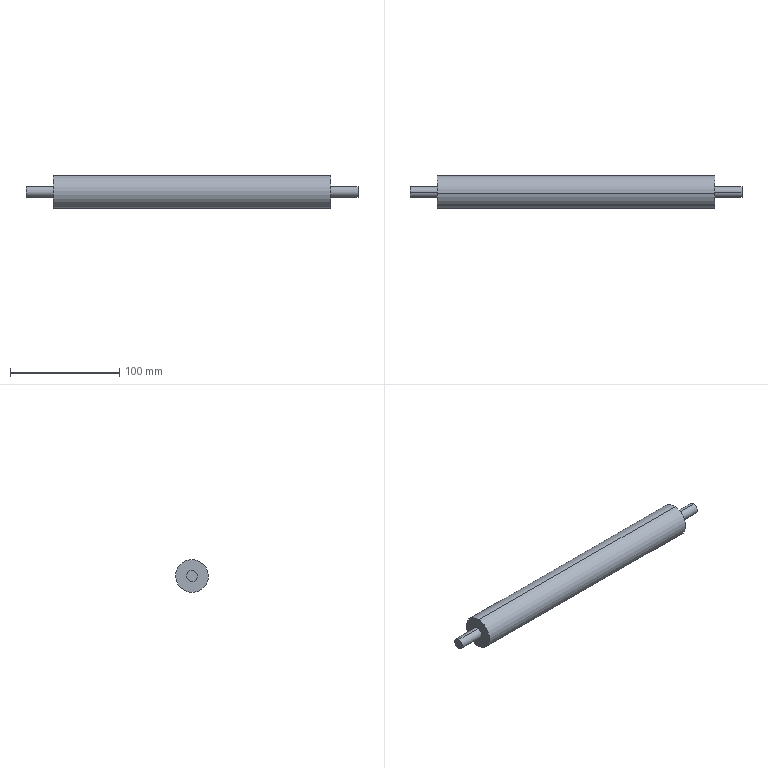Component | SolidWorks | Part5-1 | 1 solid | 10 faces | box 304 x 30 x 30 mm | volume 183469 mm3 | cylinder 6 | plane 4 | commonest cylinder face diameters 10 x4 30 x2
build123d program:
from build123d import *

# Parameters (mm, degrees)
SKETCH1_R           = 5
BOSS_EXTRUDE1_DEPTH = 152
SKETCH2_R           = 15
BOSS_EXTRUDE2_DEPTH = 127


with BuildPart() as part:
    # Sketch1 → Boss-Extrude1 (new, symmetric)
    with BuildSketch(Plane.XY):
        with Locations((-94.809, 415)):
            Circle(SKETCH1_R)
    extrude(amount=BOSS_EXTRUDE1_DEPTH, both=True)

    # Sketch2 → Boss-Extrude2 (add, symmetric)
    with BuildSketch(Plane.XY):
        with Locations((-94.809, 415)):
            Circle(SKETCH2_R)
    extrude(amount=BOSS_EXTRUDE2_DEPTH, both=True)


solid = part.part

# Placed as in the assembly
solid = solid.moved(Location((0, 0, -210.206), (0, 90, 0)))
STEP:
#1=COLOUR_RGB('',0.7922,0.8196,0.9333);
#2=FILL_AREA_STYLE_COLOUR('',#1);
#3=FILL_AREA_STYLE('',(#2));
#4=SURFACE_STYLE_FILL_AREA(#3);
#5=SURFACE_SIDE_STYLE('',(#4));
#6=SURFACE_STYLE_USAGE(.BOTH.,#5);
#7=PRESENTATION_STYLE_ASSIGNMENT((#6));
#8=CARTESIAN_POINT('',(-5.,16.355,-4.739));
#9=VERTEX_POINT('',#8);
#10=CARTESIAN_POINT('',(-5.,16.322,-4.347));
#11=VERTEX_POINT('',#10);
#12=CARTESIAN_POINT('',(-5.,16.339,-4.543));
#13=DIRECTION('',(1.,0.,0.));
#14=DIRECTION('',(0.,0.08341,-0.9965));
#15=AXIS2_PLACEMENT_3D('',#12,#13,#14);
#16=CIRCLE('',#15,0.1969);
#17=EDGE_CURVE('',#9,#11,#16,.T.);
#18=ORIENTED_EDGE('',*,*,#17,.F.);
#19=CARTESIAN_POINT('',(-5.984,16.355,-4.739));
#20=VERTEX_POINT('',#19);
#21=CARTESIAN_POINT('',(5.984,16.355,-4.739));
#22=DIRECTION('',(-1.,0.,0.));
#23=VECTOR('',#22,39.37);
#24=LINE('',#21,#23);
#25=EDGE_CURVE('',#9,#20,#24,.T.);
#26=ORIENTED_EDGE('',*,*,#25,.T.);
#27=CARTESIAN_POINT('',(-5.984,16.322,-4.347));
#28=VERTEX_POINT('',#27);
#29=CARTESIAN_POINT('',(-5.984,16.339,-4.543));
#30=DIRECTION('',(1.,0.,0.));
#31=DIRECTION('',(0.,0.08341,-0.9965));
#32=AXIS2_PLACEMENT_3D('',#29,#30,#31);
#33=CIRCLE('',#32,0.1969);
#34=EDGE_CURVE('',#20,#28,#33,.T.);
#35=ORIENTED_EDGE('',*,*,#34,.T.);
#36=CARTESIAN_POINT('',(5.984,16.322,-4.347));
#37=DIRECTION('',(-1.,0.,0.));
#38=VECTOR('',#37,39.37);
#39=LINE('',#36,#38);
#40=EDGE_CURVE('',#11,#28,#39,.T.);
#41=ORIENTED_EDGE('',*,*,#40,.F.);
#42=EDGE_LOOP('',(#18,#26,#35,#41));
#43=FACE_OUTER_BOUND('',#42,.T.);
#44=CARTESIAN_POINT('',(5.984,16.339,-4.543));
#45=DIRECTION('',(-1.,0.,0.));
#46=DIRECTION('',(0.,-0.08341,0.9965));
#47=AXIS2_PLACEMENT_3D('',#44,#45,#46);
#48=CYLINDRICAL_SURFACE('',#47,0.1969);
#49=ADVANCED_FACE('',(#43),#48,.T.);
#50=CARTESIAN_POINT('',(5.,16.388,-5.132));
#51=VERTEX_POINT('',#50);
#52=CARTESIAN_POINT('',(5.,16.289,-3.955));
#53=VERTEX_POINT('',#52);
#54=CARTESIAN_POINT('',(5.,16.339,-4.543));
#55=DIRECTION('',(1.,0.,0.));
#56=DIRECTION('',(0.,0.08341,-0.9965));
#57=AXIS2_PLACEMENT_3D('',#54,#55,#56);
#58=CIRCLE('',#57,0.5906);
#59=EDGE_CURVE('',#51,#53,#58,.T.);
#60=ORIENTED_EDGE('',*,*,#59,.F.);
#61=CARTESIAN_POINT('',(-5.,16.388,-5.132));
#62=VERTEX_POINT('',#61);
#63=CARTESIAN_POINT('',(5.,16.388,-5.132));
#64=DIRECTION('',(-1.,0.,0.));
#65=VECTOR('',#64,39.37);
#66=LINE('',#63,#65);
#67=EDGE_CURVE('',#51,#62,#66,.T.);
#68=ORIENTED_EDGE('',*,*,#67,.T.);
#69=CARTESIAN_POINT('',(-5.,16.289,-3.955));
#70=VERTEX_POINT('',#69);
#71=CARTESIAN_POINT('',(-5.,16.339,-4.543));
#72=DIRECTION('',(1.,0.,0.));
#73=DIRECTION('',(0.,0.08341,-0.9965));
#74=AXIS2_PLACEMENT_3D('',#71,#72,#73);
#75=CIRCLE('',#74,0.5906);
#76=EDGE_CURVE('',#62,#70,#75,.T.);
#77=ORIENTED_EDGE('',*,*,#76,.T.);
#78=CARTESIAN_POINT('',(5.,16.289,-3.955));
#79=DIRECTION('',(-1.,0.,0.));
#80=VECTOR('',#79,39.37);
#81=LINE('',#78,#80);
#82=EDGE_CURVE('',#53,#70,#81,.T.);
#83=ORIENTED_EDGE('',*,*,#82,.F.);
#84=EDGE_LOOP('',(#60,#68,#77,#83));
#85=FACE_OUTER_BOUND('',#84,.T.);
#86=CARTESIAN_POINT('',(5.,16.339,-4.543));
#87=DIRECTION('',(-1.,0.,0.));
#88=DIRECTION('',(0.,-0.08341,0.9965));
#89=AXIS2_PLACEMENT_3D('',#86,#87,#88);
#90=CYLINDRICAL_SURFACE('',#89,0.5906);
#91=ADVANCED_FACE('',(#85),#90,.T.);
#92=CARTESIAN_POINT('',(5.984,16.355,-4.739));
#93=VERTEX_POINT('',#92);
#94=CARTESIAN_POINT('',(5.984,16.322,-4.347));
#95=VERTEX_POINT('',#94);
#96=CARTESIAN_POINT('',(5.984,16.339,-4.543));
#97=DIRECTION('',(1.,0.,0.));
#98=DIRECTION('',(0.,0.08341,-0.9965));
#99=AXIS2_PLACEMENT_3D('',#96,#97,#98);
#100=CIRCLE('',#99,0.1969);
#101=EDGE_CURVE('',#93,#95,#100,.T.);
#102=ORIENTED_EDGE('',*,*,#101,.F.);
#103=CARTESIAN_POINT('',(5.,16.355,-4.739));
#104=VERTEX_POINT('',#103);
#105=CARTESIAN_POINT('',(5.984,16.355,-4.739));
#106=DIRECTION('',(-1.,0.,0.));
#107=VECTOR('',#106,39.37);
#108=LINE('',#105,#107);
#109=EDGE_CURVE('',#93,#104,#108,.T.);
#110=ORIENTED_EDGE('',*,*,#109,.T.);
#111=CARTESIAN_POINT('',(5.,16.322,-4.347));
#112=VERTEX_POINT('',#111);
#113=CARTESIAN_POINT('',(5.,16.339,-4.543));
#114=DIRECTION('',(1.,0.,0.));
#115=DIRECTION('',(0.,0.08341,-0.9965));
#116=AXIS2_PLACEMENT_3D('',#113,#114,#115);
#117=CIRCLE('',#116,0.1969);
#118=EDGE_CURVE('',#104,#112,#117,.T.);
#119=ORIENTED_EDGE('',*,*,#118,.T.);
#120=CARTESIAN_POINT('',(5.984,16.322,-4.347));
#121=DIRECTION('',(-1.,0.,0.));
#122=VECTOR('',#121,39.37);
#123=LINE('',#120,#122);
#124=EDGE_CURVE('',#95,#112,#123,.T.);
#125=ORIENTED_EDGE('',*,*,#124,.F.);
#126=EDGE_LOOP('',(#102,#110,#119,#125));
#127=FACE_OUTER_BOUND('',#126,.T.);
#128=CARTESIAN_POINT('',(5.984,16.339,-4.543));
#129=DIRECTION('',(-1.,0.,0.));
#130=DIRECTION('',(0.,-0.08341,0.9965));
#131=AXIS2_PLACEMENT_3D('',#128,#129,#130);
#132=CYLINDRICAL_SURFACE('',#131,0.1969);
#133=ADVANCED_FACE('',(#127),#132,.T.);
#134=ORIENTED_EDGE('',*,*,#109,.F.);
#135=CARTESIAN_POINT('',(5.984,16.339,-4.543));
#136=DIRECTION('',(1.,0.,0.));
#137=DIRECTION('',(0.,0.08341,-0.9965));
#138=AXIS2_PLACEMENT_3D('',#135,#136,#137);
#139=CIRCLE('',#138,0.1969);
#140=EDGE_CURVE('',#95,#93,#139,.T.);
#141=ORIENTED_EDGE('',*,*,#140,.F.);
#142=ORIENTED_EDGE('',*,*,#124,.T.);
#143=CARTESIAN_POINT('',(5.,16.339,-4.543));
#144=DIRECTION('',(1.,0.,0.));
#145=DIRECTION('',(0.,0.08341,-0.9965));
#146=AXIS2_PLACEMENT_3D('',#143,#144,#145);
#147=CIRCLE('',#146,0.1969);
#148=EDGE_CURVE('',#112,#104,#147,.T.);
#149=ORIENTED_EDGE('',*,*,#148,.T.);
#150=EDGE_LOOP('',(#134,#141,#142,#149));
#151=FACE_OUTER_BOUND('',#150,.T.);
#152=CARTESIAN_POINT('',(5.984,16.339,-4.543));
#153=DIRECTION('',(-1.,0.,0.));
#154=DIRECTION('',(0.,-0.08341,0.9965));
#155=AXIS2_PLACEMENT_3D('',#152,#153,#154);
#156=CYLINDRICAL_SURFACE('',#155,0.1969);
#157=ADVANCED_FACE('',(#151),#156,.T.);
#158=ORIENTED_EDGE('',*,*,#140,.T.);
#159=ORIENTED_EDGE('',*,*,#101,.T.);
#160=EDGE_LOOP('',(#158,#159));
#161=FACE_OUTER_BOUND('',#160,.T.);
#162=CARTESIAN_POINT('',(5.984,16.339,-4.543));
#163=DIRECTION('',(1.,0.,0.));
#164=DIRECTION('',(0.,0.08341,-0.9965));
#165=AXIS2_PLACEMENT_3D('',#162,#163,#164);
#166=PLANE('',#165);
#167=ADVANCED_FACE('',(#161),#166,.T.);
#168=ORIENTED_EDGE('',*,*,#67,.F.);
#169=CARTESIAN_POINT('',(5.,16.339,-4.543));
#170=DIRECTION('',(1.,0.,0.));
#171=DIRECTION('',(0.,0.08341,-0.9965));
#172=AXIS2_PLACEMENT_3D('',#169,#170,#171);
#173=CIRCLE('',#172,0.5906);
#174=EDGE_CURVE('',#53,#51,#173,.T.);
#175=ORIENTED_EDGE('',*,*,#174,.F.);
#176=ORIENTED_EDGE('',*,*,#82,.T.);
#177=CARTESIAN_POINT('',(-5.,16.339,-4.543));
#178=DIRECTION('',(1.,0.,0.));
#179=DIRECTION('',(0.,0.08341,-0.9965));
#180=AXIS2_PLACEMENT_3D('',#177,#178,#179);
#181=CIRCLE('',#180,0.5906);
#182=EDGE_CURVE('',#70,#62,#181,.T.);
#183=ORIENTED_EDGE('',*,*,#182,.T.);
#184=EDGE_LOOP('',(#168,#175,#176,#183));
#185=FACE_OUTER_BOUND('',#184,.T.);
#186=CARTESIAN_POINT('',(5.,16.339,-4.543));
#187=DIRECTION('',(-1.,0.,0.));
#188=DIRECTION('',(0.,-0.08341,0.9965));
#189=AXIS2_PLACEMENT_3D('',#186,#187,#188);
#190=CYLINDRICAL_SURFACE('',#189,0.5906);
#191=ADVANCED_FACE('',(#185),#190,.T.);
#192=ORIENTED_EDGE('',*,*,#148,.F.);
#193=ORIENTED_EDGE('',*,*,#118,.F.);
#194=EDGE_LOOP('',(#192,#193));
#195=FACE_BOUND('',#194,.T.);
#196=ORIENTED_EDGE('',*,*,#174,.T.);
#197=ORIENTED_EDGE('',*,*,#59,.T.);
#198=EDGE_LOOP('',(#196,#197));
#199=FACE_OUTER_BOUND('',#198,.T.);
#200=CARTESIAN_POINT('',(5.,16.339,-4.543));
#201=DIRECTION('',(1.,0.,0.));
#202=DIRECTION('',(0.,0.08341,-0.9965));
#203=AXIS2_PLACEMENT_3D('',#200,#201,#202);
#204=PLANE('',#203);
#205=ADVANCED_FACE('',(#195,#199),#204,.T.);
#206=CARTESIAN_POINT('',(-5.,16.339,-4.543));
#207=DIRECTION('',(1.,0.,0.));
#208=DIRECTION('',(0.,0.08341,-0.9965));
#209=AXIS2_PLACEMENT_3D('',#206,#207,#208);
#210=CIRCLE('',#209,0.1969);
#211=EDGE_CURVE('',#11,#9,#210,.T.);
#212=ORIENTED_EDGE('',*,*,#211,.T.);
#213=ORIENTED_EDGE('',*,*,#17,.T.);
#214=EDGE_LOOP('',(#212,#213));
#215=FACE_BOUND('',#214,.T.);
#216=ORIENTED_EDGE('',*,*,#182,.F.);
#217=ORIENTED_EDGE('',*,*,#76,.F.);
#218=EDGE_LOOP('',(#216,#217));
#219=FACE_OUTER_BOUND('',#218,.T.);
#220=CARTESIAN_POINT('',(-5.,16.339,-4.543));
#221=DIRECTION('',(1.,0.,0.));
#222=DIRECTION('',(0.,0.08341,-0.9965));
#223=AXIS2_PLACEMENT_3D('',#220,#221,#222);
#224=PLANE('',#223);
#225=ADVANCED_FACE('',(#215,#219),#224,.F.);
#226=CARTESIAN_POINT('',(-5.984,16.339,-4.543));
#227=DIRECTION('',(1.,0.,0.));
#228=DIRECTION('',(0.,0.08341,-0.9965));
#229=AXIS2_PLACEMENT_3D('',#226,#227,#228);
#230=CIRCLE('',#229,0.1969);
#231=EDGE_CURVE('',#28,#20,#230,.T.);
#232=ORIENTED_EDGE('',*,*,#231,.F.);
#233=ORIENTED_EDGE('',*,*,#34,.F.);
#234=EDGE_LOOP('',(#232,#233));
#235=FACE_OUTER_BOUND('',#234,.T.);
#236=CARTESIAN_POINT('',(-5.984,16.339,-4.543));
#237=DIRECTION('',(1.,0.,0.));
#238=DIRECTION('',(0.,0.08341,-0.9965));
#239=AXIS2_PLACEMENT_3D('',#236,#237,#238);
#240=PLANE('',#239);
#241=ADVANCED_FACE('',(#235),#240,.F.);
#242=ORIENTED_EDGE('',*,*,#25,.F.);
#243=ORIENTED_EDGE('',*,*,#211,.F.);
#244=ORIENTED_EDGE('',*,*,#40,.T.);
#245=ORIENTED_EDGE('',*,*,#231,.T.);
#246=EDGE_LOOP('',(#242,#243,#244,#245));
#247=FACE_OUTER_BOUND('',#246,.T.);
#248=CARTESIAN_POINT('',(5.984,16.339,-4.543));
#249=DIRECTION('',(-1.,0.,0.));
#250=DIRECTION('',(0.,-0.08341,0.9965));
#251=AXIS2_PLACEMENT_3D('',#248,#249,#250);
#252=CYLINDRICAL_SURFACE('',#251,0.1969);
#253=ADVANCED_FACE('',(#247),#252,.T.);
#254=CLOSED_SHELL('',(#49,#91,#133,#157,#167,#191,#205,#225,#241,#253));
#255=MANIFOLD_SOLID_BREP('',#254);
#256=STYLED_ITEM('',(#7),#255);
#257=(LENGTH_UNIT()NAMED_UNIT(*)SI_UNIT($,.METRE.));
#258=LENGTH_MEASURE_WITH_UNIT(LENGTH_MEASURE(0.0254),#257);
#259=DIMENSIONAL_EXPONENTS(1.,0.,0.,0.,0.,0.,0.);
#260=(CONVERSION_BASED_UNIT('',#258)LENGTH_UNIT()NAMED_UNIT(#259));
#261=UNCERTAINTY_MEASURE_WITH_UNIT(LENGTH_MEASURE(0.00001),#260,'','');
#262=(NAMED_UNIT(*)PLANE_ANGLE_UNIT()SI_UNIT($,.RADIAN.));
#263=(NAMED_UNIT(*)SI_UNIT($,.STERADIAN.)SOLID_ANGLE_UNIT());
#264=(GEOMETRIC_REPRESENTATION_CONTEXT(3)GLOBAL_UNCERTAINTY_ASSIGNED_CONTEXT((#261))GLOBAL_UNIT_ASSIGNED_CONTEXT((#260,#262,#263))REPRESENTATION_CONTEXT('',''));
#265=MECHANICAL_DESIGN_GEOMETRIC_PRESENTATION_REPRESENTATION('',(#256),#264);
#266=CARTESIAN_POINT('',(0.,0.,0.));
#267=DIRECTION('',(0.,0.,1.));
#268=DIRECTION('',(1.,0.,0.));
#269=AXIS2_PLACEMENT_3D('',#266,#267,#268);
#270=(LENGTH_UNIT()NAMED_UNIT(*)SI_UNIT($,.METRE.));
#271=LENGTH_MEASURE_WITH_UNIT(LENGTH_MEASURE(0.0254),#270);
#272=DIMENSIONAL_EXPONENTS(1.,0.,0.,0.,0.,0.,0.);
#273=(CONVERSION_BASED_UNIT('',#271)LENGTH_UNIT()NAMED_UNIT(#272));
#274=UNCERTAINTY_MEASURE_WITH_UNIT(LENGTH_MEASURE(0.00001),#273,'','');
#275=(NAMED_UNIT(*)PLANE_ANGLE_UNIT()SI_UNIT($,.RADIAN.));
#276=(NAMED_UNIT(*)SI_UNIT($,.STERADIAN.)SOLID_ANGLE_UNIT());
#277=(GEOMETRIC_REPRESENTATION_CONTEXT(3)GLOBAL_UNCERTAINTY_ASSIGNED_CONTEXT((#274))GLOBAL_UNIT_ASSIGNED_CONTEXT((#273,#275,#276))REPRESENTATION_CONTEXT('',''));
#278=ADVANCED_BREP_SHAPE_REPRESENTATION('',(#255,#269),#277);
#279=PRESENTATION_LAYER_ASSIGNMENT('','',(#256));